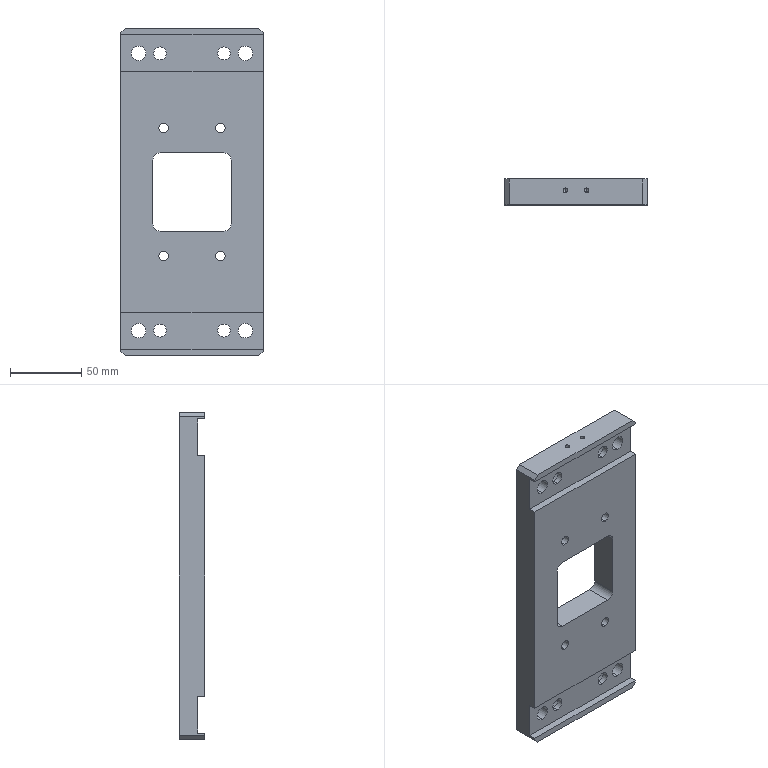Component | SolidWorks | 300-05-1 | 1 solid | 86 faces | box 100 x 18 x 230 mm | volume 317926 mm3 | cylinder 48 | plane 26 | cone 12 | commonest cylinder face diameters 3.3 x8 6.8 x8 15 x8 9 x8 10.2 x8 8 x4 10 x4 | material 45
build123d program:
from build123d import *

# Parameters (mm, degrees)
SKETCH1_W                  = 230
SKETCH1_H                  = 100
BOSS_EXTRUDE1_DEPTH        = 9
SKETCH2_W                  = 26
SKETCH2_H                  = 100
CUT_EXTRUDE1_DEPTH         = 5
SKETCH7_W                  = 55
SKETCH7_H                  = 55
CUT_EXTRUDE2_DEPTH         = 127.685
FILLET1_R                  = 5
CHAMFER1_SIZE              = 3
M4_TAPPED_HOLE1_AT_2_COUNT = 2
M4_TAPPED_HOLE1_AT_2_PITCH = 15


with BuildPart() as part:
    # Sketch1 → Boss-Extrude1 (new, symmetric)
    with BuildSketch(Plane.XY):
        Rectangle(SKETCH1_W, SKETCH1_H)
    extrude(amount=BOSS_EXTRUDE1_DEPTH, both=True)

    # Sketch2 → Cut-Extrude1 (cut)
    with BuildSketch(Plane.XY.offset(9)):
        with Locations((97.5, 0)):
            Rectangle(SKETCH2_W, SKETCH2_H)
    cut_extrude1 = extrude(amount=-CUT_EXTRUDE1_DEPTH, mode=Mode.SUBTRACT)

    # Mirror1: Cut-Extrude1 across plane
    add(cut_extrude1.mirror(Plane(origin=(0, 0, 0), x_dir=(0, 0, 1), z_dir=(1, 0, 0))), mode=Mode.SUBTRACT)

    # Sketch4 → M12 Tapped Hole1 (revolve, cut)
    with BuildSketch(Plane(origin=(-97.5, 37.5, -9), x_dir=(0, 1, 0), z_dir=(1, 0, 0))):
        Polygon((0, 0), (0, 32.314), (5.1, 29.25), (5.1, 0), align=None)
    m12_tapped_hole1 = revolve(axis=Axis((-97.5, 37.5, -15.35), (0, 0, 1)), mode=Mode.SUBTRACT)

    # Sketch6 → Hole Size _According to_ Type of Hexagon (revolve, cut)
    with BuildSketch(Plane(origin=(-97.5, 22.5, -9), x_dir=(0, 1, 0), z_dir=(1, 0, 0))):
        Polygon((0, 0), (0, 31.954), (4.5, 29.25), (4.5, 9), (7.5, 9), (7.5, 0), align=None)
    hole_size_according_to_type_of_hexagon = revolve(axis=Axis((-97.5, 22.5, -15.35), (0, 0, 1)), mode=Mode.SUBTRACT)

    # Mirror2: M12 Tapped Hole1, Hole Size _According to_ Type of Hexagon across plane
    add(m12_tapped_hole1.mirror(Plane.ZX), mode=Mode.SUBTRACT)
    add(hole_size_according_to_type_of_hexagon.mirror(Plane.ZX), mode=Mode.SUBTRACT)

    # Mirror3: M12 Tapped Hole1, Hole Size _According to_ Type of Hexagon across plane
    add(m12_tapped_hole1.mirror(Plane(origin=(0, 0, 0), x_dir=(0, 0, 1), z_dir=(1, 0, 0))), mode=Mode.SUBTRACT)
    add(hole_size_according_to_type_of_hexagon.mirror(Plane(origin=(0, 0, 0), x_dir=(0, 0, 1), z_dir=(1, 0, 0))), mode=Mode.SUBTRACT)

    # Mirror3 copy 1 sketch → Mirror3 copy 1 (revolve, cut)
    with BuildSketch(Plane(origin=(97.5, -37.5, -9), x_dir=(0, -1, 0), z_dir=(-1, 0, 0))):
        Polygon((0, 0), (0, 32.314), (5.1, 29.25), (5.1, 0), align=None)
    revolve(axis=Axis((97.5, -37.5, -15.35), (0, 0, 1)), mode=Mode.SUBTRACT)

    # Mirror3 copy 2 sketch → Mirror3 copy 2 (revolve, cut)
    with BuildSketch(Plane(origin=(97.5, -22.5, -9), x_dir=(0, -1, 0), z_dir=(-1, 0, 0))):
        Polygon((0, 0), (0, 31.954), (4.5, 29.25), (4.5, 9), (7.5, 9), (7.5, 0), align=None)
    revolve(axis=Axis((97.5, -22.5, -15.35), (0, 0, 1)), mode=Mode.SUBTRACT)

    # Sketch7 → Cut-Extrude2 (cut, through all)
    with BuildSketch(Plane(origin=(0, 0, -9), x_dir=(-1, 0, 0), z_dir=(0, 0, -1))):
        Rectangle(SKETCH7_W, SKETCH7_H)
    extrude(amount=-CUT_EXTRUDE2_DEPTH, mode=Mode.SUBTRACT)

    # Fillet1
    fillet1_edges = [part.edges().sort_by_distance(p)[0] for p in [
        (-27.5, 27.5, 0),
        (-27.5, -27.5, 0),
        (27.5, -27.5, 0),
        (27.5, 27.5, 0),
    ]]
    fillet(fillet1_edges, radius=FILLET1_R)

    # Sketch9 → M8 Tapped Hole1 (revolve, cut)
    with BuildSketch(Plane(origin=(-45, 20, -9), x_dir=(0, 1, 0), z_dir=(1, 0, 0))):
        Polygon((0, 0), (0, 21.793), (3.4, 19.75), (3.4, 0), align=None)
    m8_tapped_hole1 = revolve(axis=Axis((-45, 20, -15.35), (0, 0, 1)), mode=Mode.SUBTRACT)

    # Sketch11 → Size mm Dowel Pin Hole1 (revolve, cut)
    with BuildSketch(Plane(origin=(-45, 0, -9), x_dir=(0, 1, 0), z_dir=(1, 0, 0))):
        Polygon((0, 0), (0, 12.403), (4, 10), (4, 0), align=None)
    size_mm_dowel_pin_hole1 = revolve(axis=Axis((-45, 0, -15.35), (0, 0, 1)), mode=Mode.SUBTRACT)

    # Mirror4: M8 Tapped Hole1 across plane
    add(m8_tapped_hole1.mirror(Plane.ZX), mode=Mode.SUBTRACT)

    # Mirror5: M8 Tapped Hole1, Size mm Dowel Pin Hole1 across plane
    add(m8_tapped_hole1.mirror(Plane(origin=(0, 0, 0), x_dir=(0, 0, 1), z_dir=(1, 0, 0))), mode=Mode.SUBTRACT)
    add(size_mm_dowel_pin_hole1.mirror(Plane(origin=(0, 0, 0), x_dir=(0, 0, 1), z_dir=(1, 0, 0))), mode=Mode.SUBTRACT)

    # Mirror5 copy 1 sketch → Mirror5 copy 1 (revolve, cut)
    with BuildSketch(Plane(origin=(45, -20, -9), x_dir=(0, -1, 0), z_dir=(-1, 0, 0))):
        Polygon((0, 0), (0, 21.793), (3.4, 19.75), (3.4, 0), align=None)
    revolve(axis=Axis((45, -20, -15.35), (0, 0, 1)), mode=Mode.SUBTRACT)

    # Chamfer1
    chamfer1_edges = [part.edges().sort_by_distance(p)[0] for p in [
        (115, -50, 0),
        (-115, -50, 0),
        (-115, 50, 0),
        (115, 50, 0),
    ]]
    chamfer(chamfer1_edges, length=CHAMFER1_SIZE)

    # Sketch13 → M4 Tapped Hole1 (revolve, cut)
    with BuildSketch(Plane(origin=(-115, -7.5, -1), x_dir=(0, 0, 1), z_dir=(0, 1, 0))):
        Polygon((0, 0), (0, 11.091), (1.65, 10.1), (1.65, 0), align=None)
    m4_tapped_hole1 = revolve(axis=Axis((-121.35, -7.5, -1), (1, 0, 0)), mode=Mode.SUBTRACT)

    # M4 Tapped Hole1 at 2: M4 Tapped Hole1 ×2
    with Locations(*[(0, i * M4_TAPPED_HOLE1_AT_2_PITCH, 0) for i in range(1, M4_TAPPED_HOLE1_AT_2_COUNT)]):
        add(m4_tapped_hole1, mode=Mode.SUBTRACT)

    # Mirror6: M4 Tapped Hole1 across plane
    add(m4_tapped_hole1.mirror(Plane(origin=(0, 0, 0), x_dir=(0, 0, 1), z_dir=(1, 0, 0))), mode=Mode.SUBTRACT)

    # Mirror6 copy 1 sketch → Mirror6 copy 1 (revolve, cut)
    with BuildSketch(Plane(origin=(115, 7.5, -1), x_dir=(0, 0, 1), z_dir=(0, 1, 0))):
        Polygon((0, 0), (0, -11.091), (1.65, -10.1), (1.65, 0), align=None)
    revolve(axis=Axis((121.35, 7.5, -1), (1, 0, 0)), mode=Mode.SUBTRACT)


solid = part.part

# Placed as in the assembly
solid = solid.moved(Location((230, 144, 0), (90, 0, 90)))